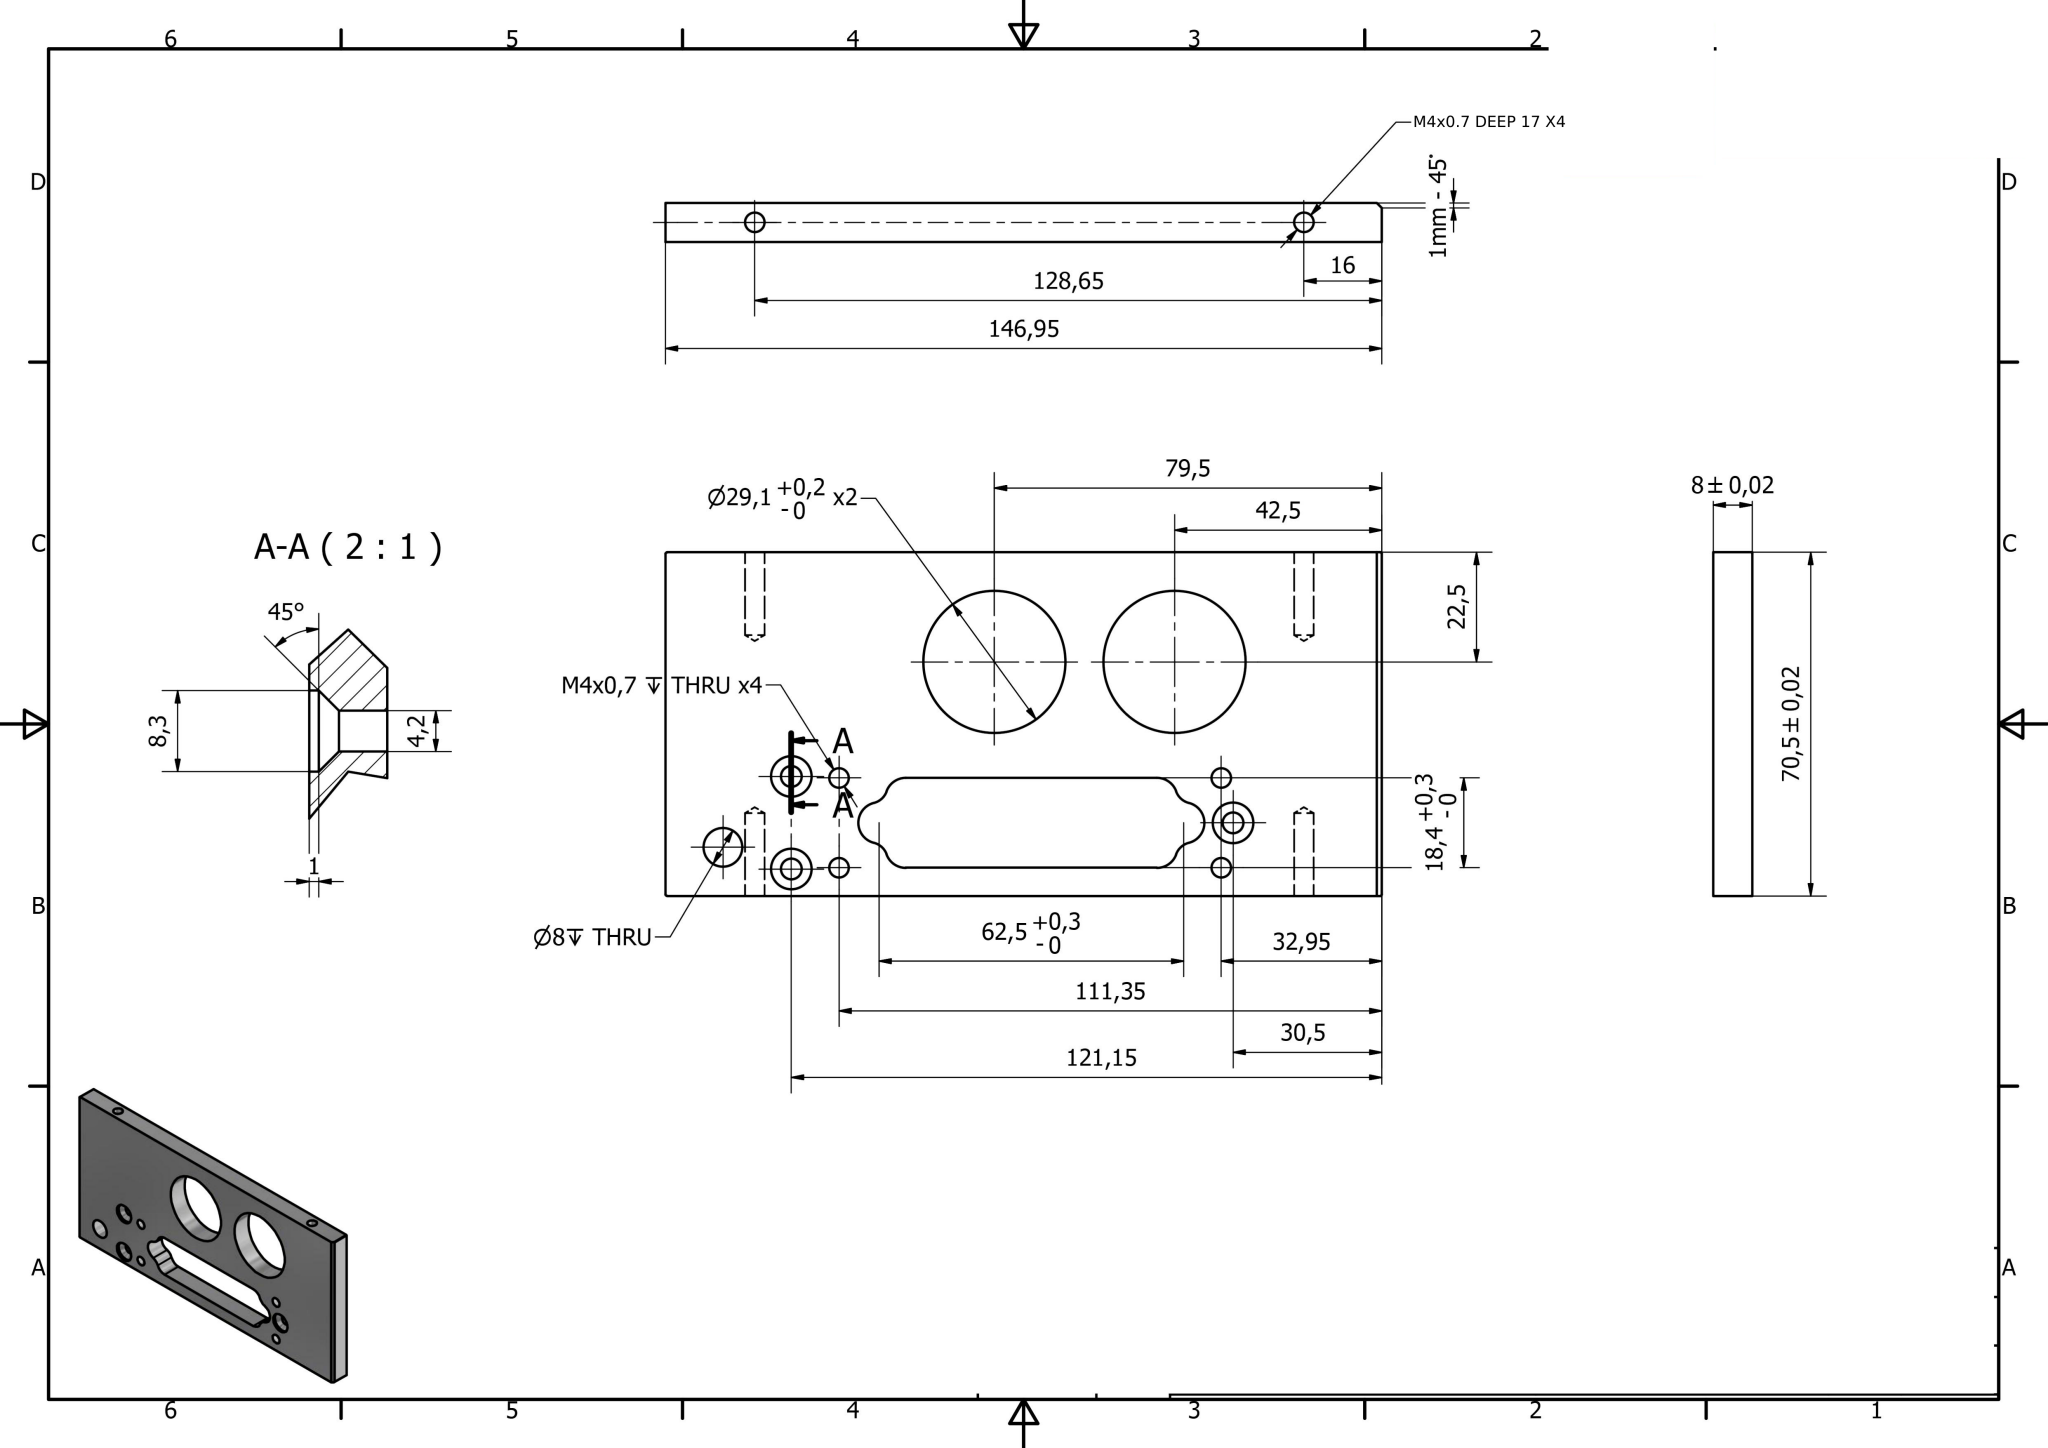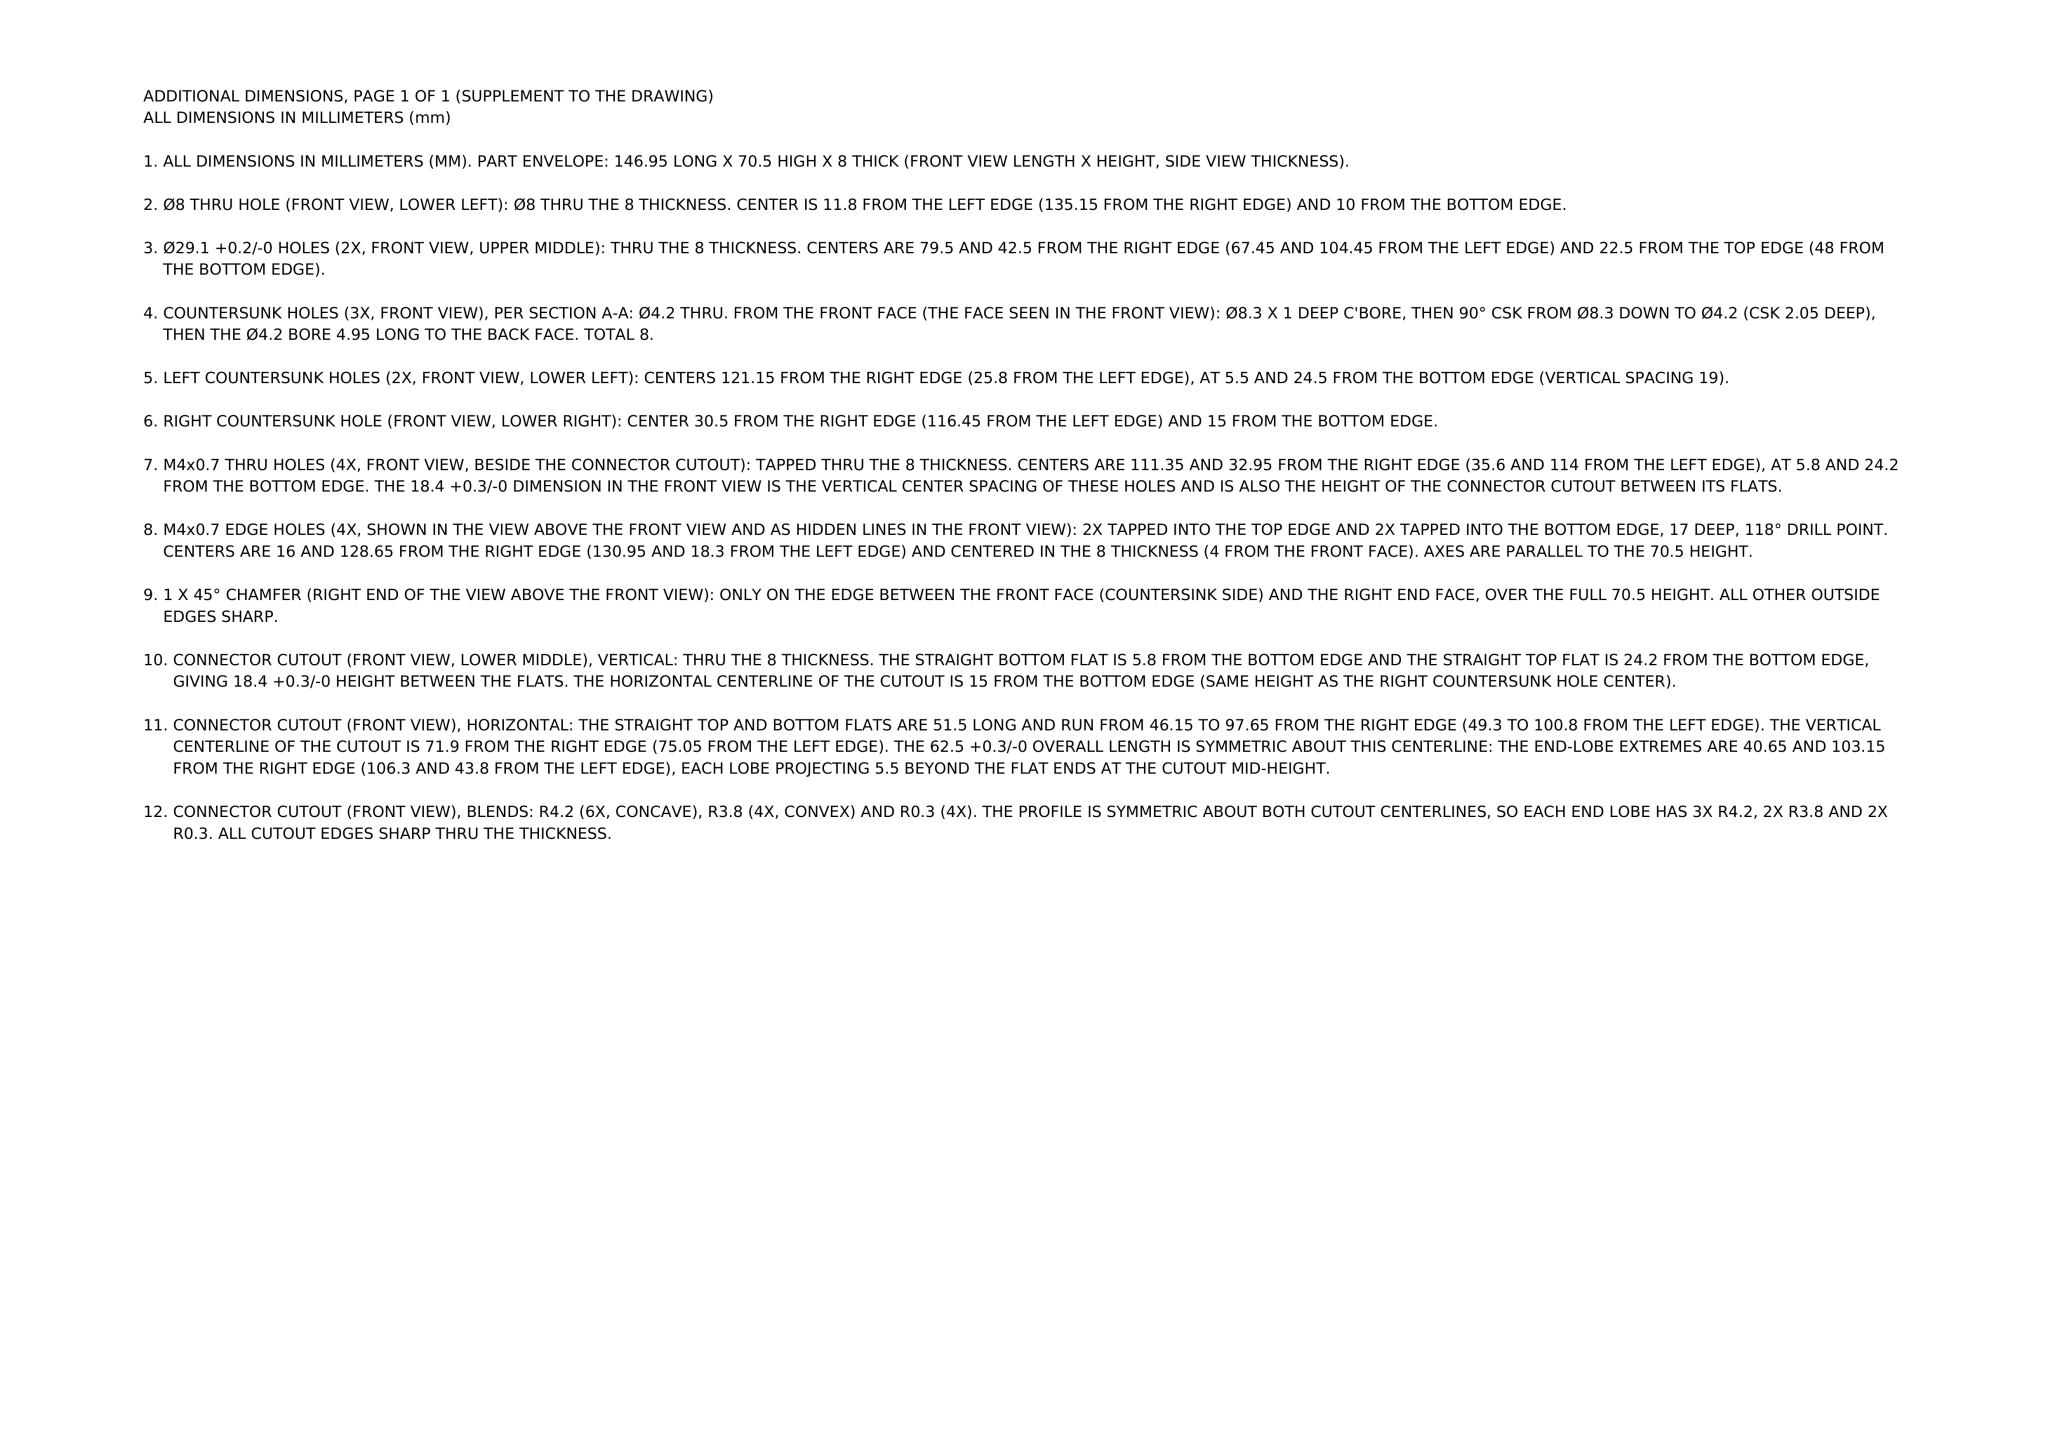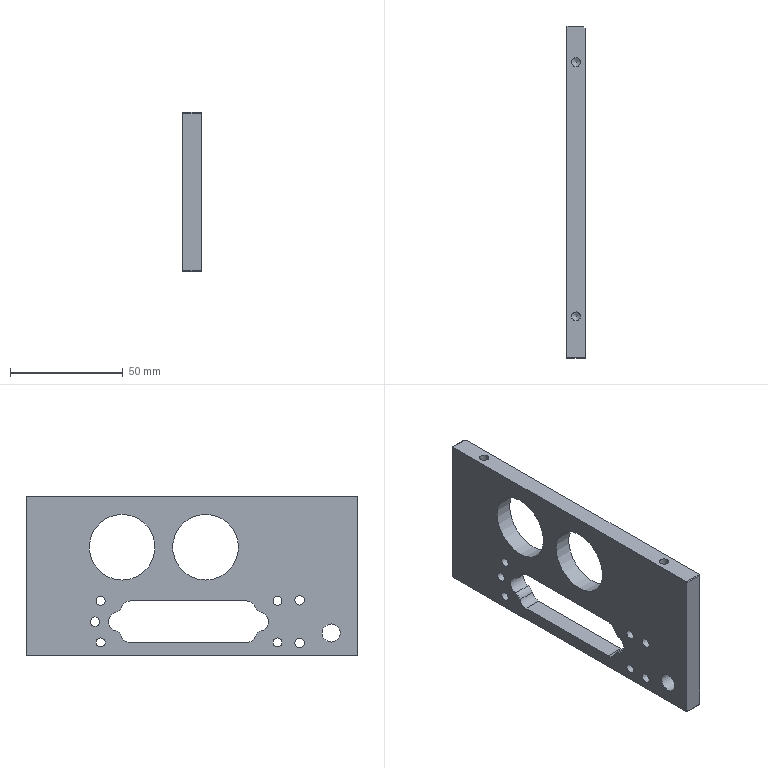Part | NX | mm | 1 solid | 47 faces | box 8 x 146.95 x 70.5 mm | volume 60604 mm3 | cylinder 31 | plane 9 | cone 7 | commonest cylinder face diameters 4 x8 8.4 x6 0.6 x4 7.6 x4 4.2 x3 8.3 x3 29.1 x2 8 x1